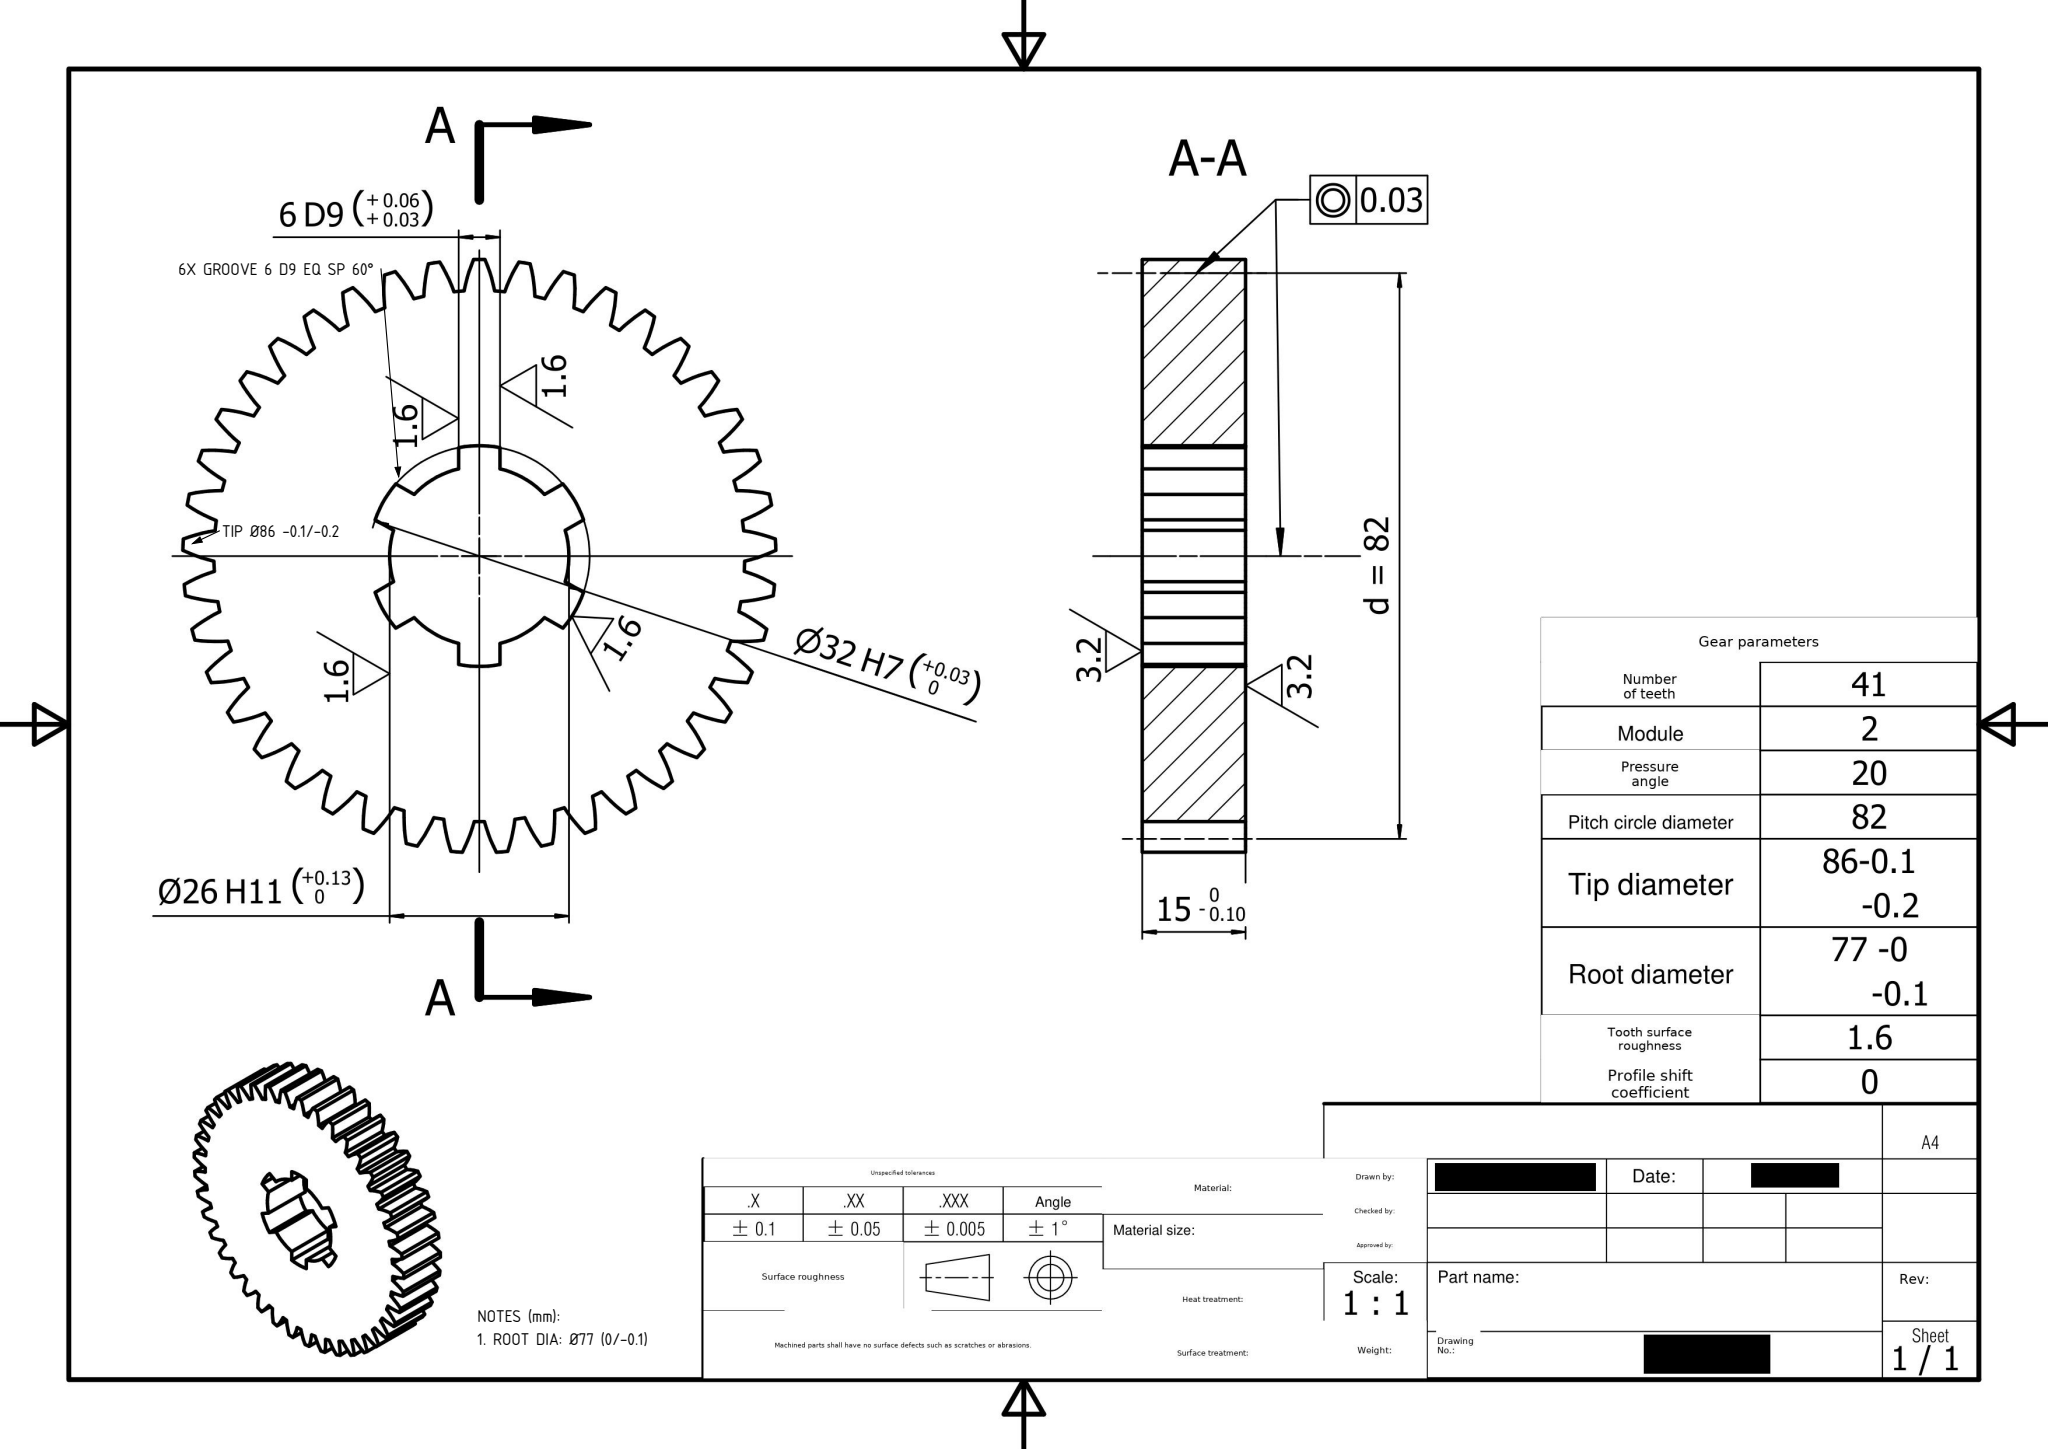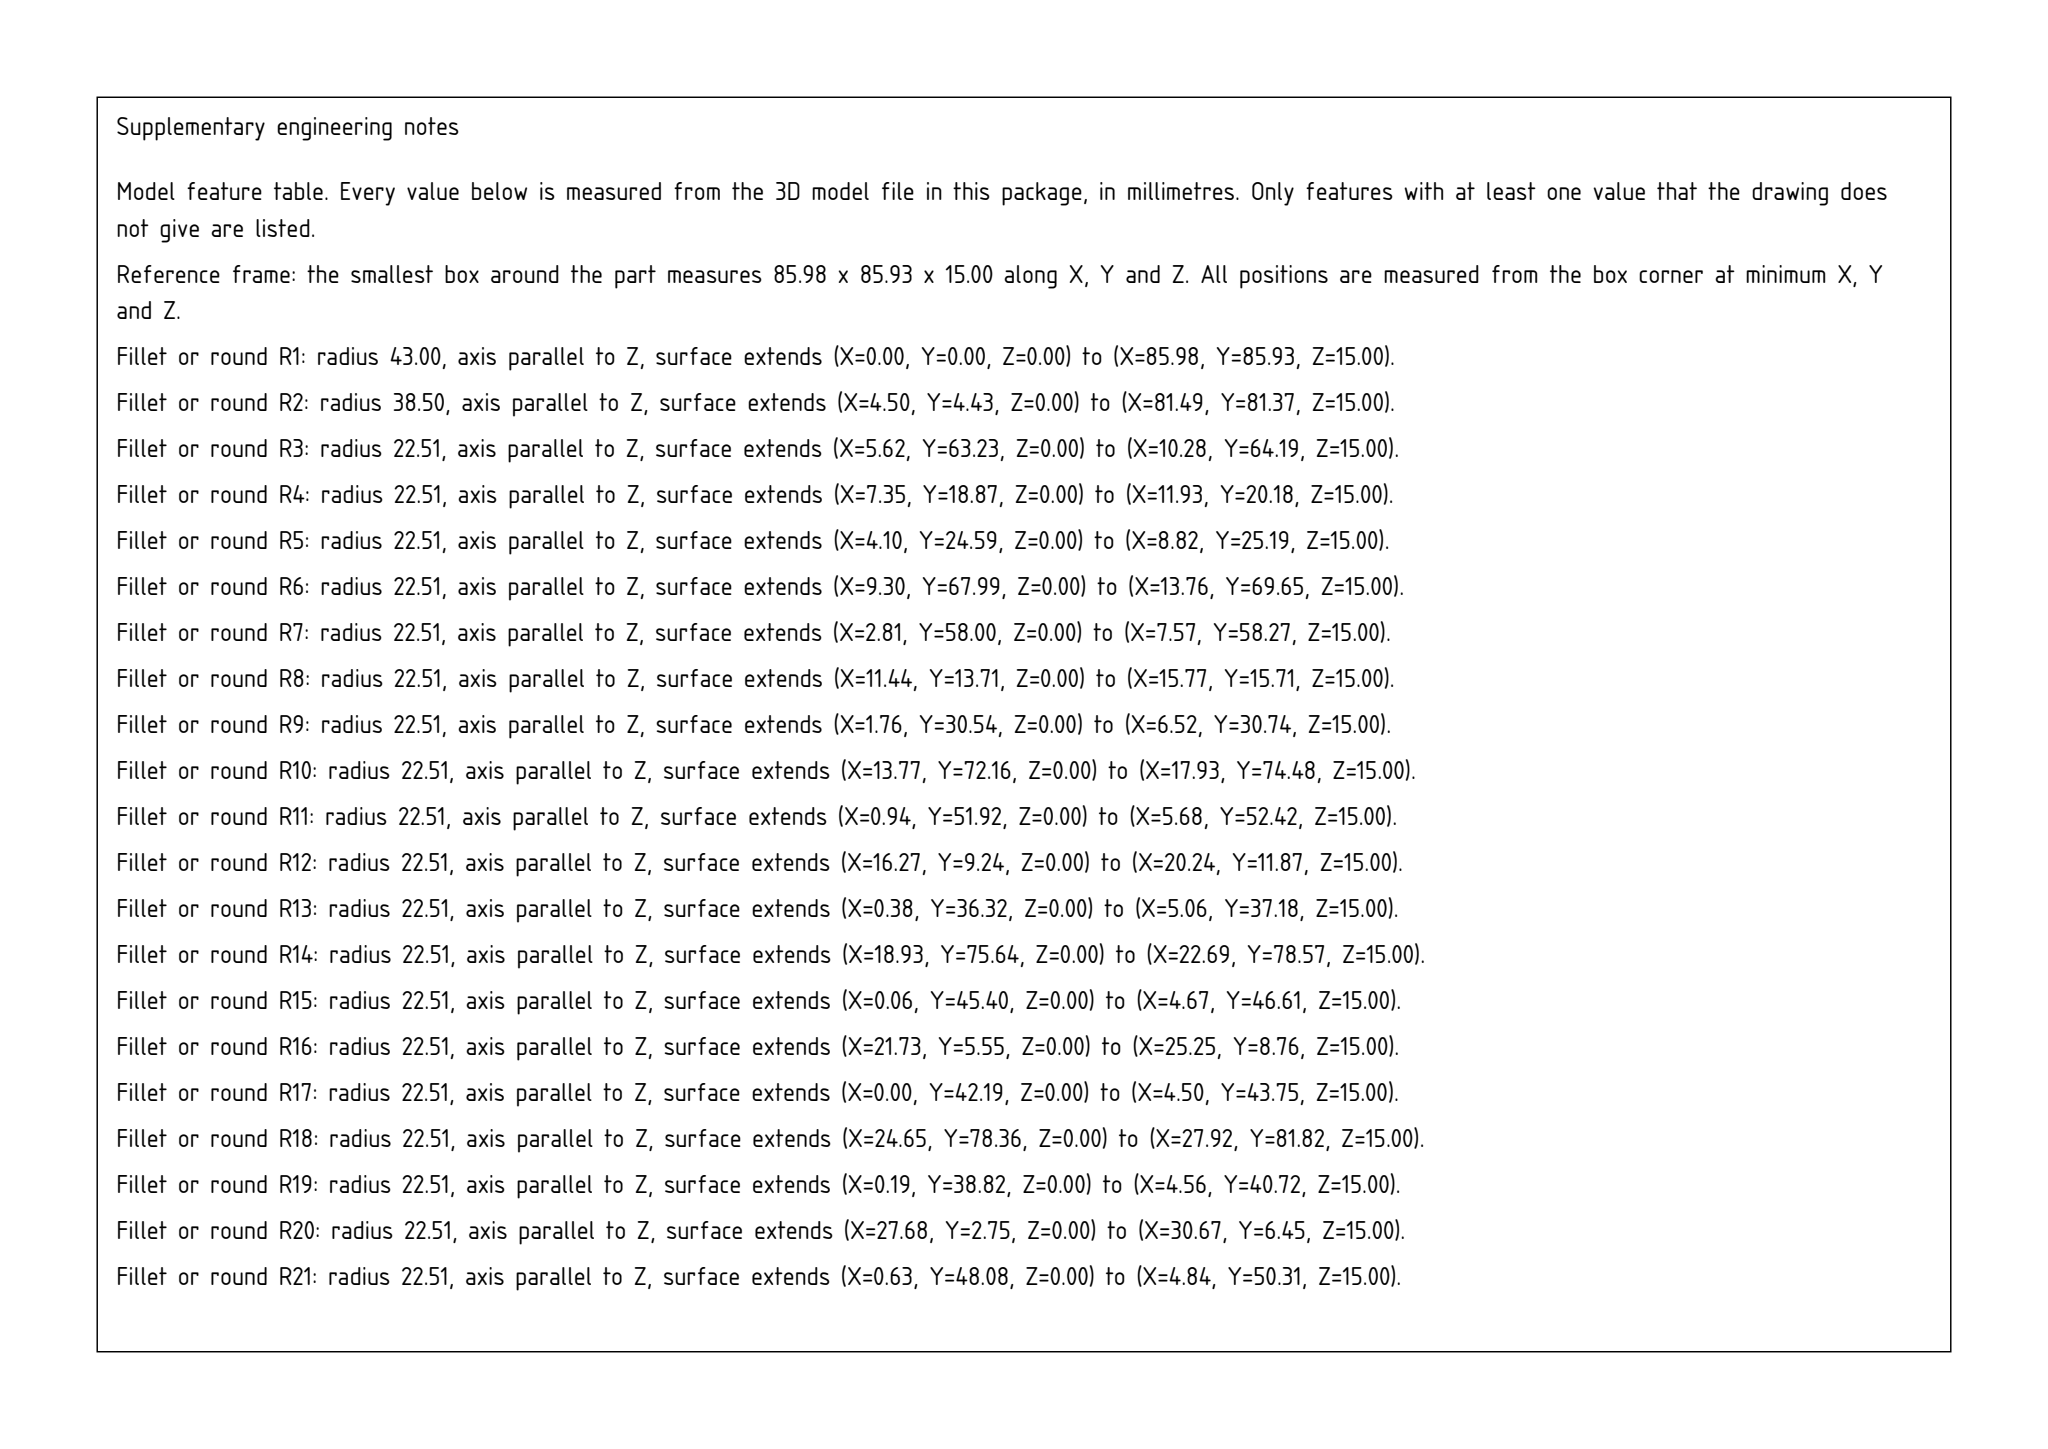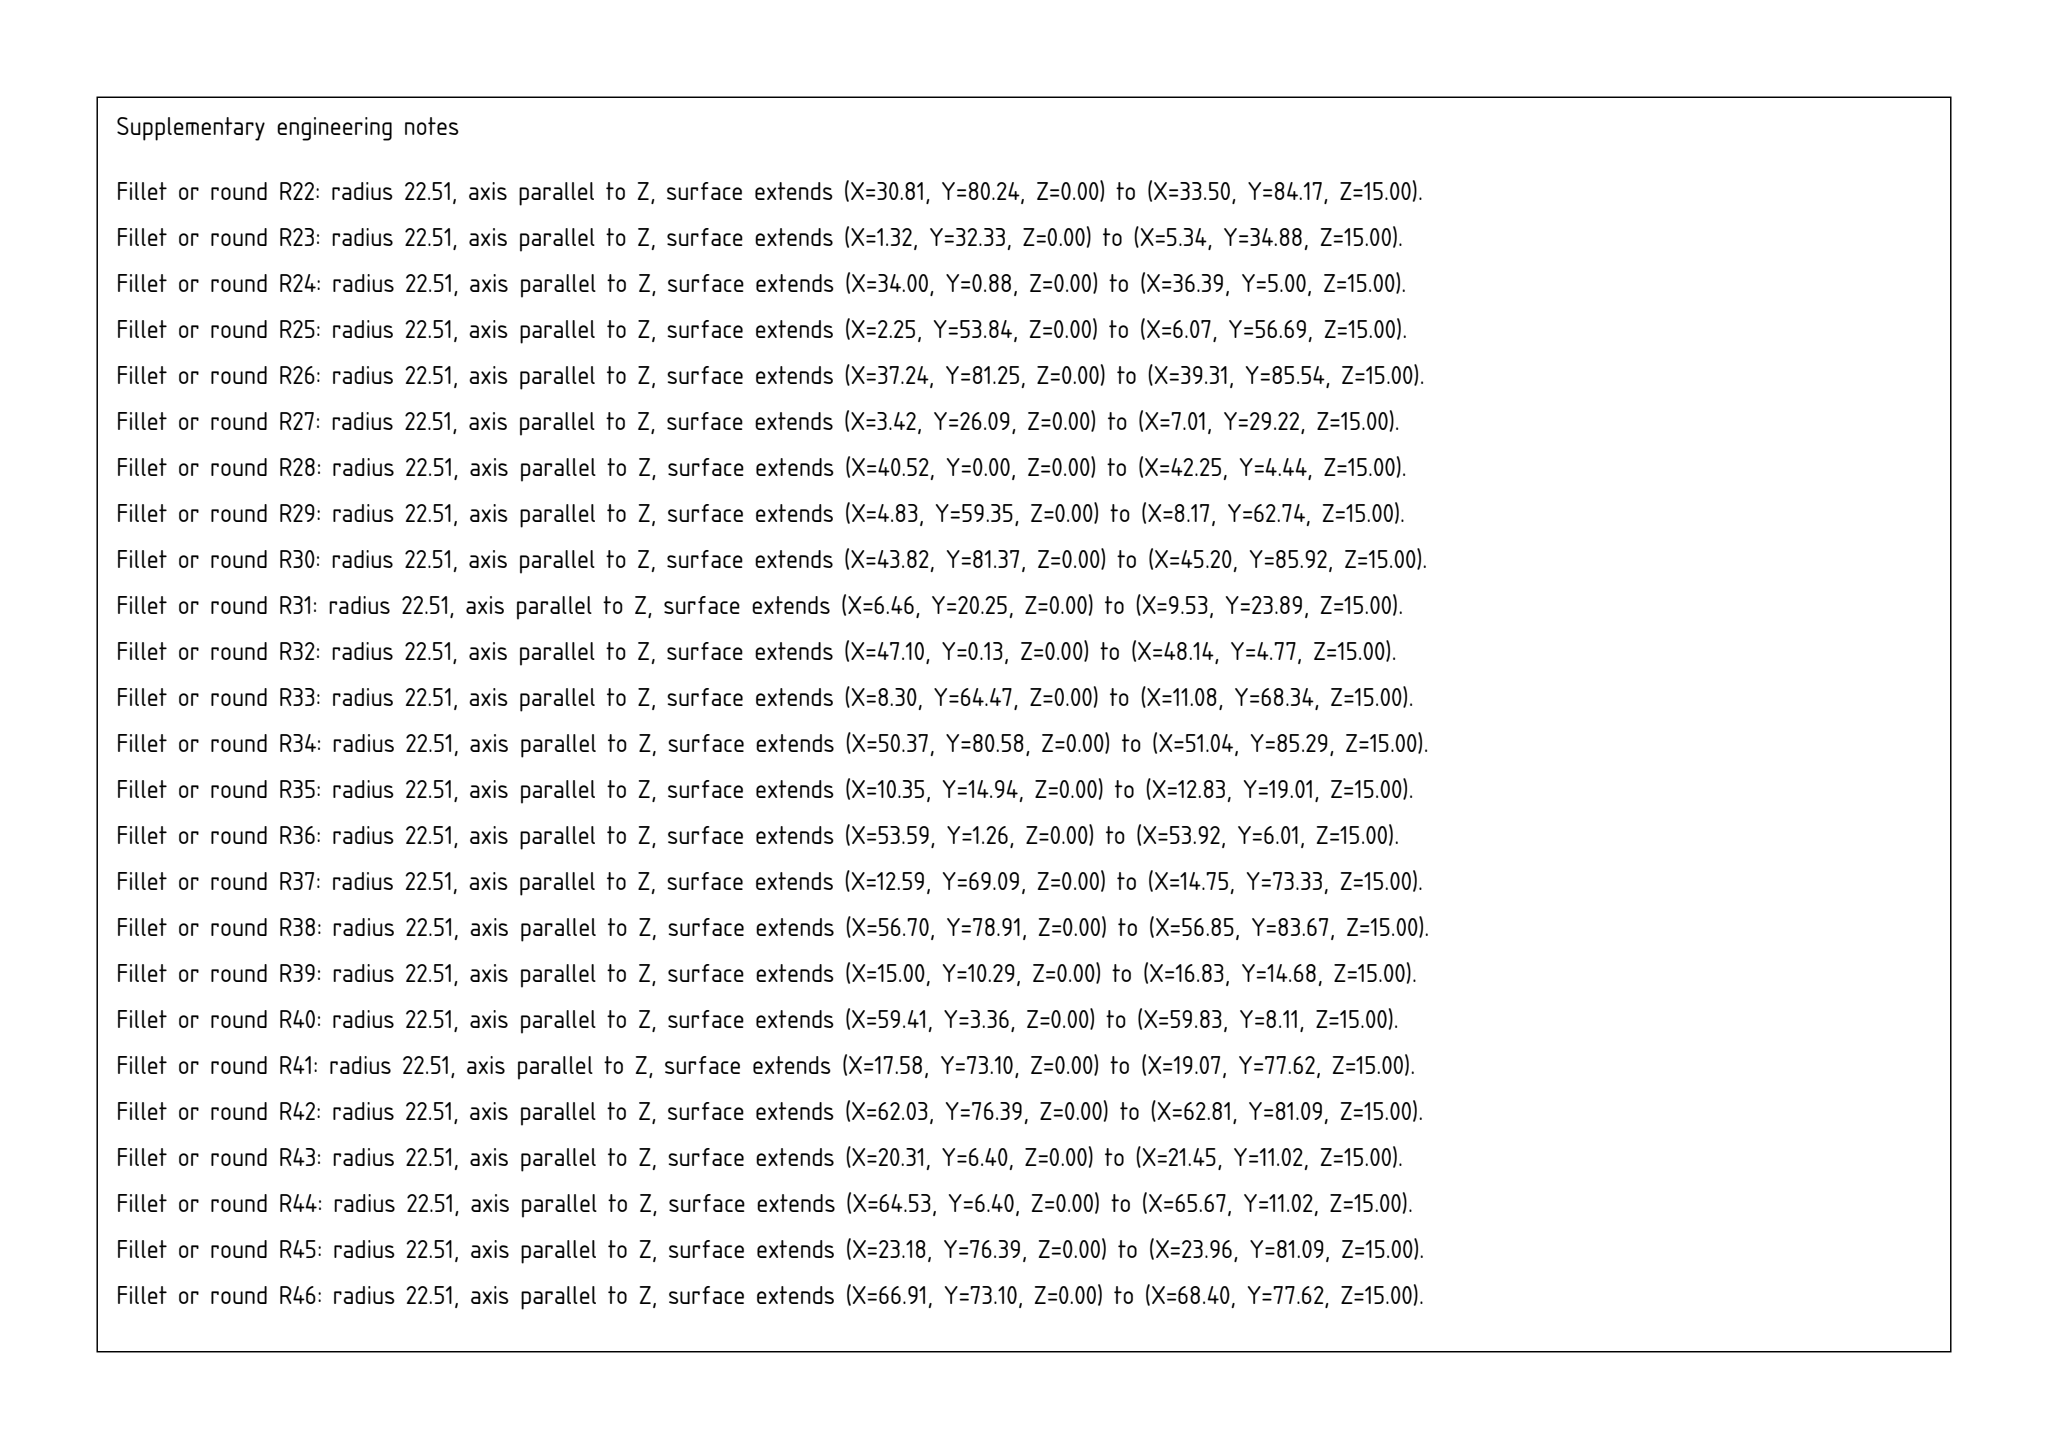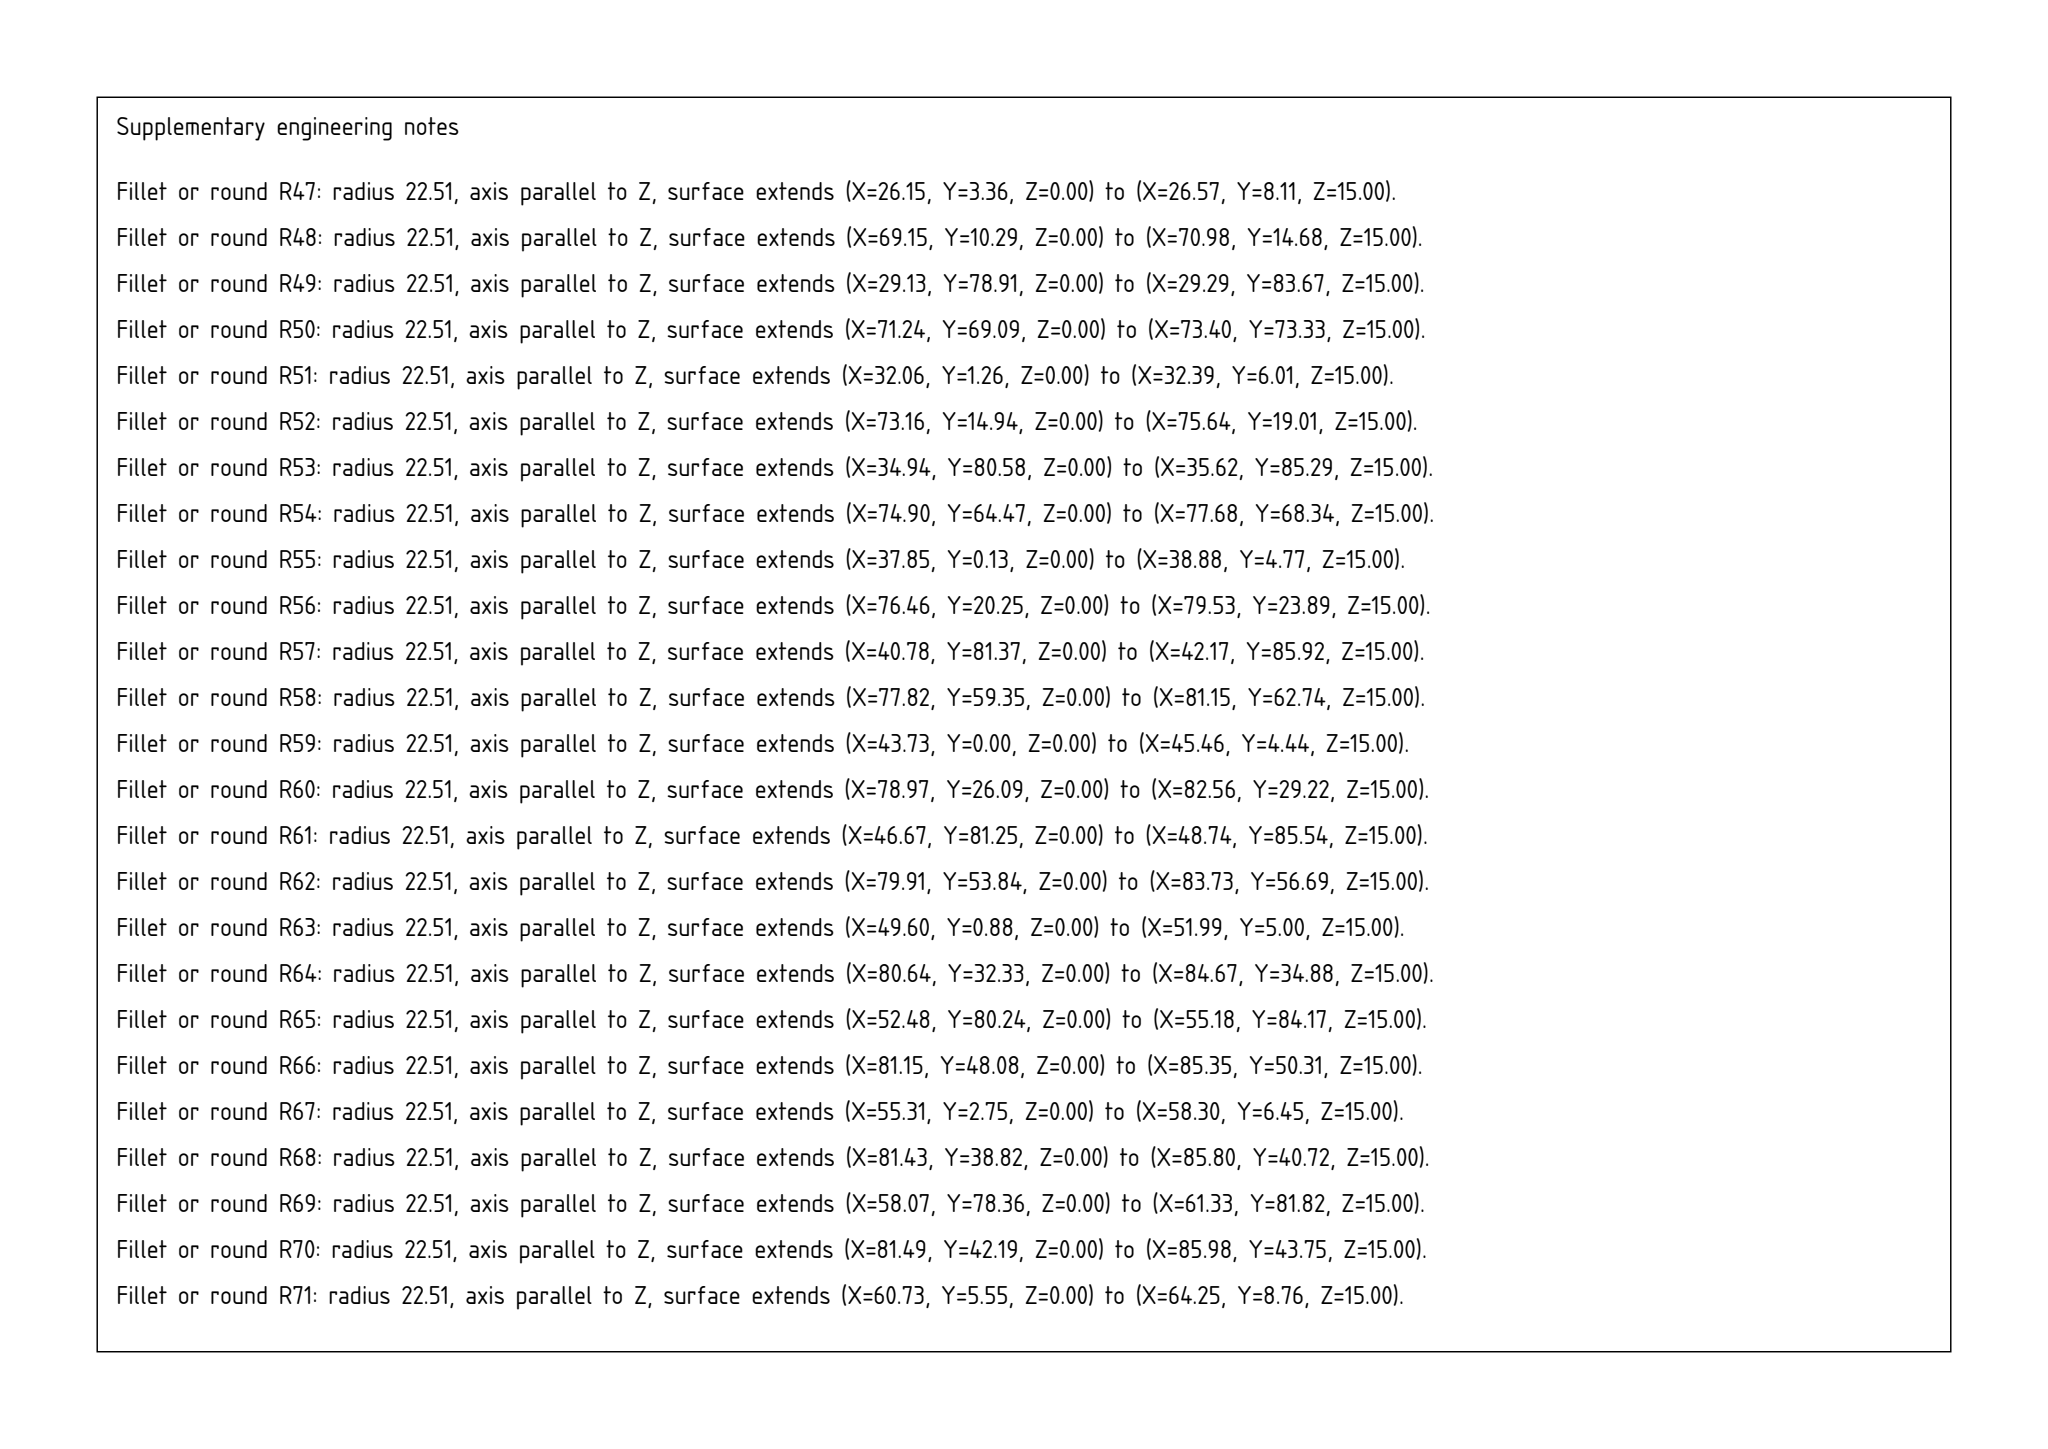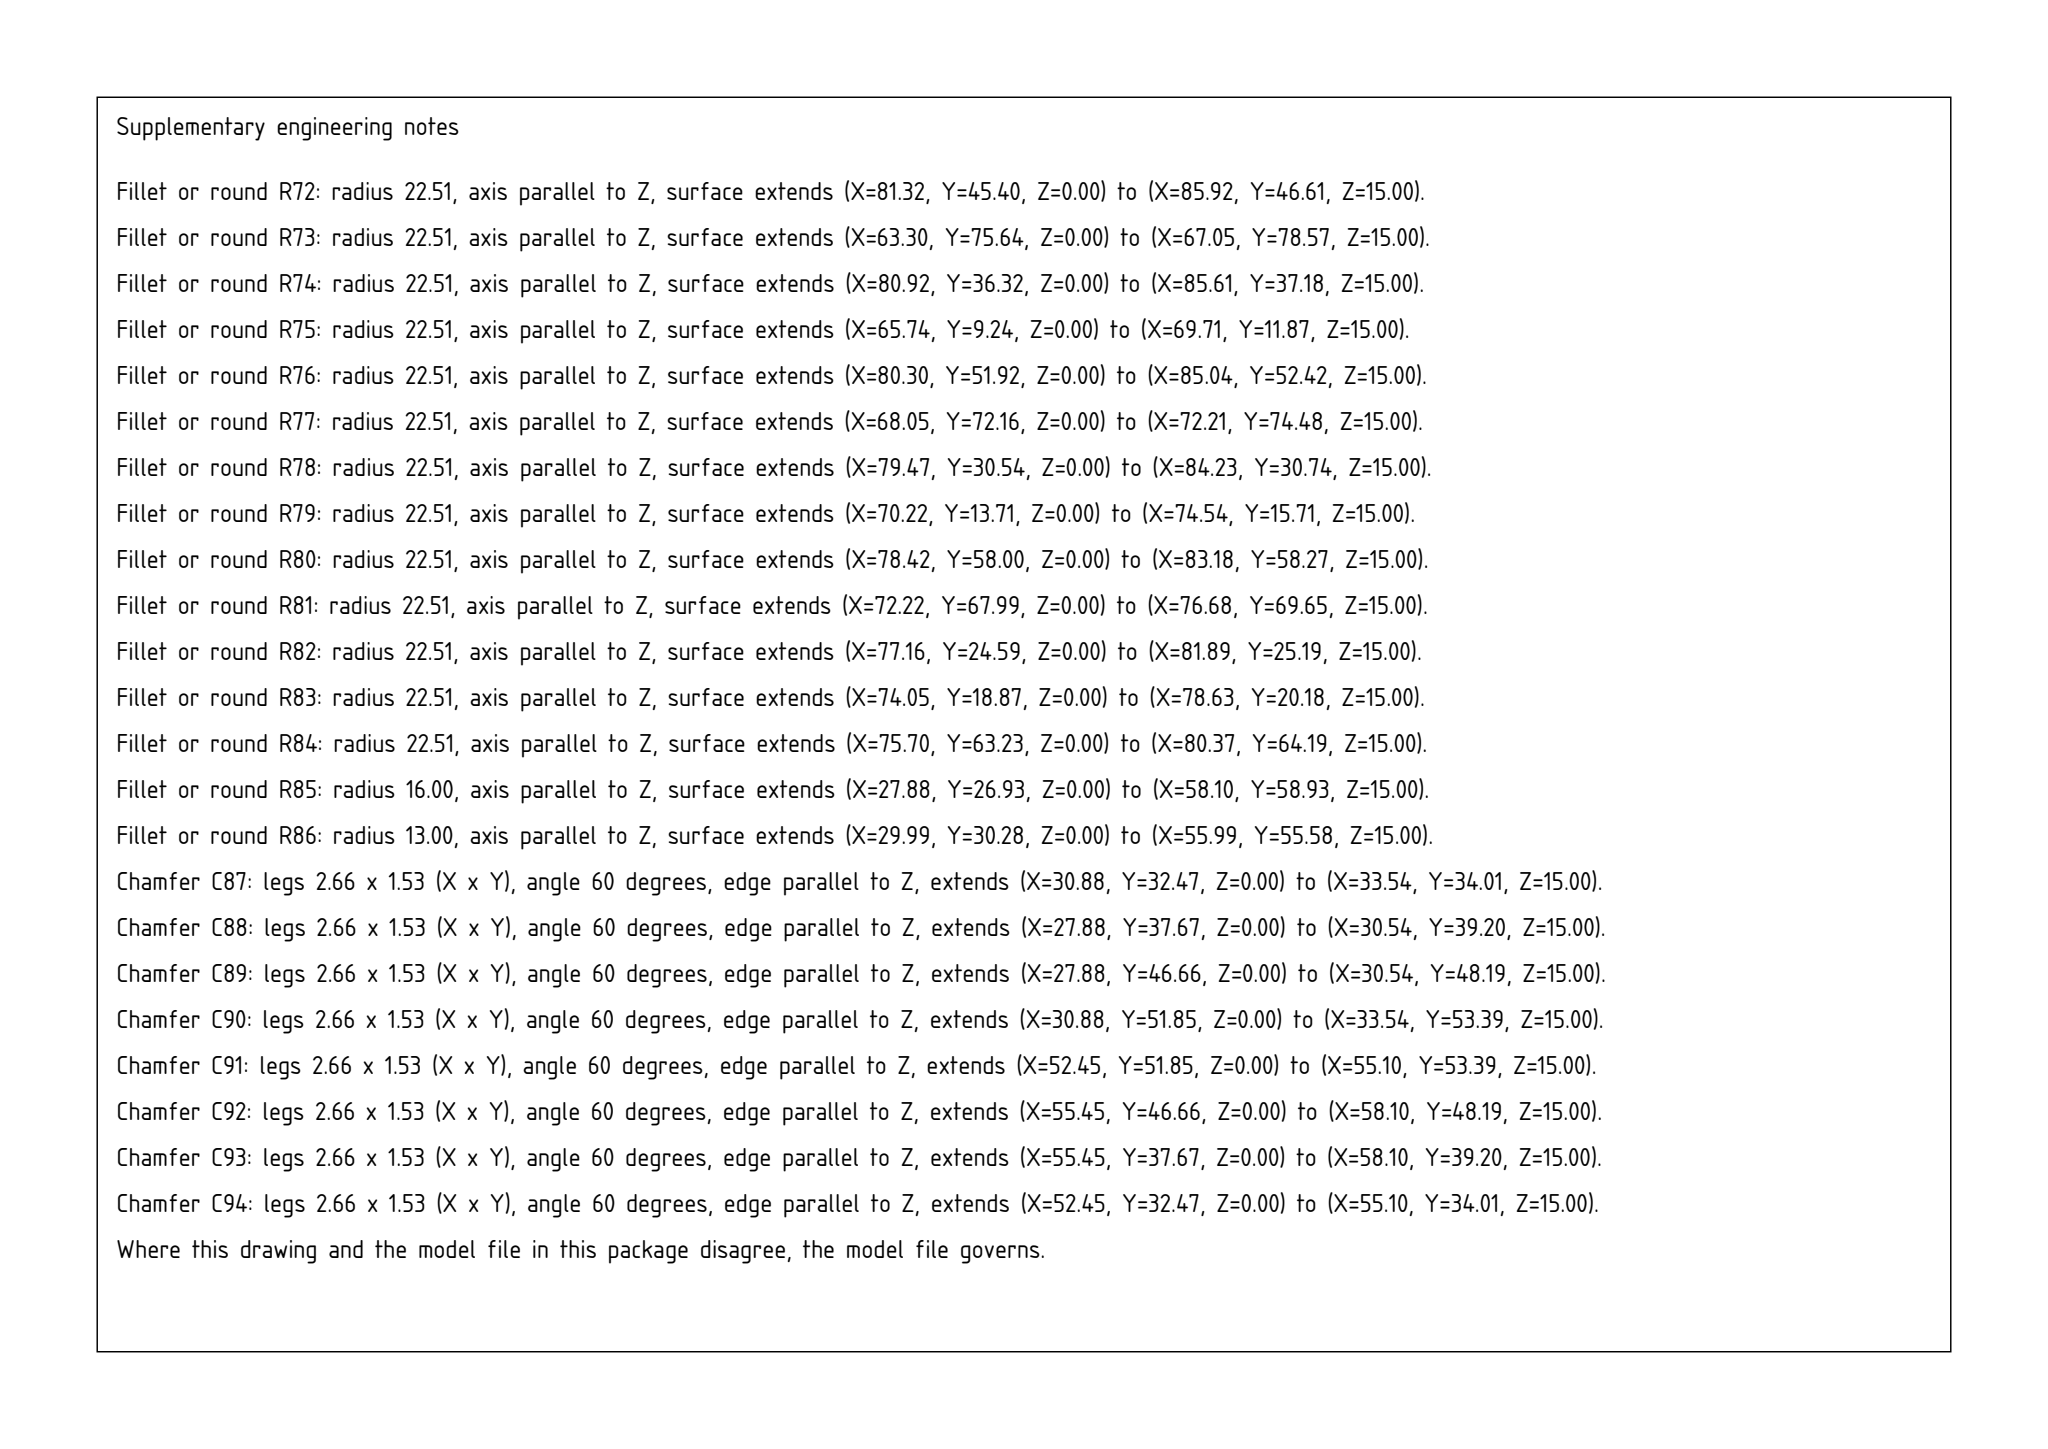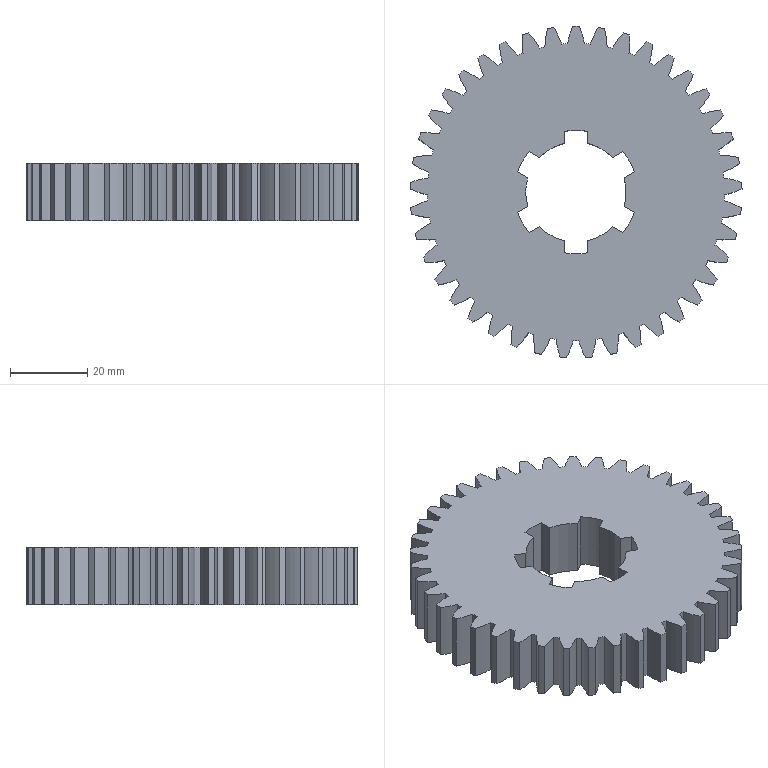Part | SolidWorks | mm | 1 solid | 194 faces | box 85.98 x 85.93 x 15 mm | volume 69140 mm3 | cylinder 180 | plane 14 | commonest cylinder face diameters 45.024 x85 86 x41 77 x41 26 x7 32 x6
Drawing notes:
6X SPLINE GROOVE 6 D9 EQ SP 60° ABOUT Ø32 H7 BORE AXIS | from the solid: 7 arcs Ø26 + 6 arcs Ø32 coaxial at (42.99,42.93); groove flanks planes x=39.99 & x=45.99 (6 wide), 6 grooves => 360/6=60° EQS
TIP DIA: Ø86 (-0.1/-0.2), MEASURES Ø85.9 MAX | from the solid: bbox_xyz 85.984 x 85.929 across tooth tips, z-axis gear
ROOT DIA: Ø77 (0/-0.1) | from the solid: m=2, z=41, pitch dia 82 => root dia 82-5=77; tooth fillet cyls r=45.024 at root